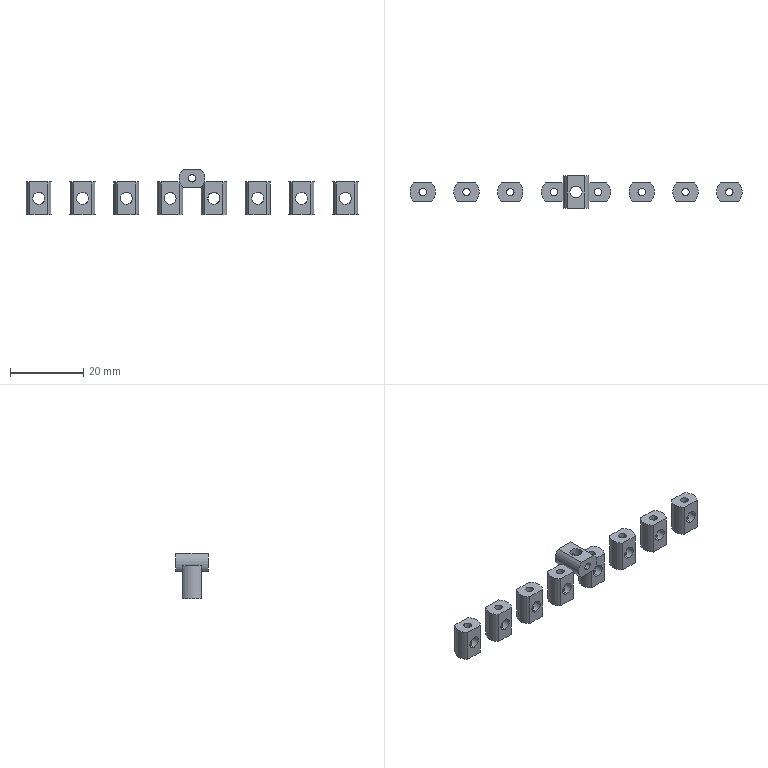CAM job | Mastercam | mm | 15 operations | part box 91 x 9 x 12.5
1. 3D High Speed (Dynamic OptiRough) | 2 - 10C
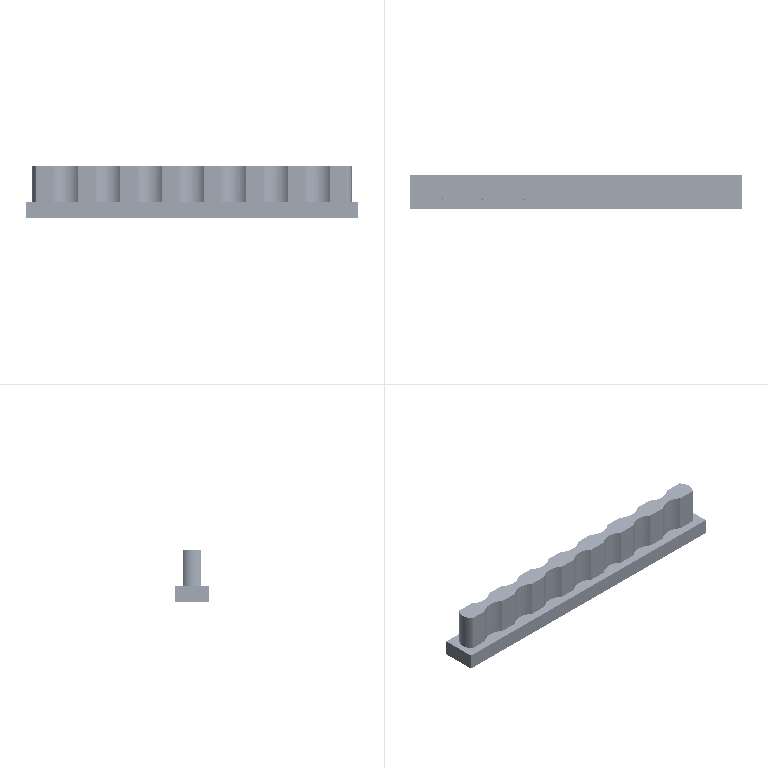2. Facing | 3 - 10J
3. 3D High Speed (Waterline rest passes) | 4 - 4C
4. Contour (2D) | 5 - 4J
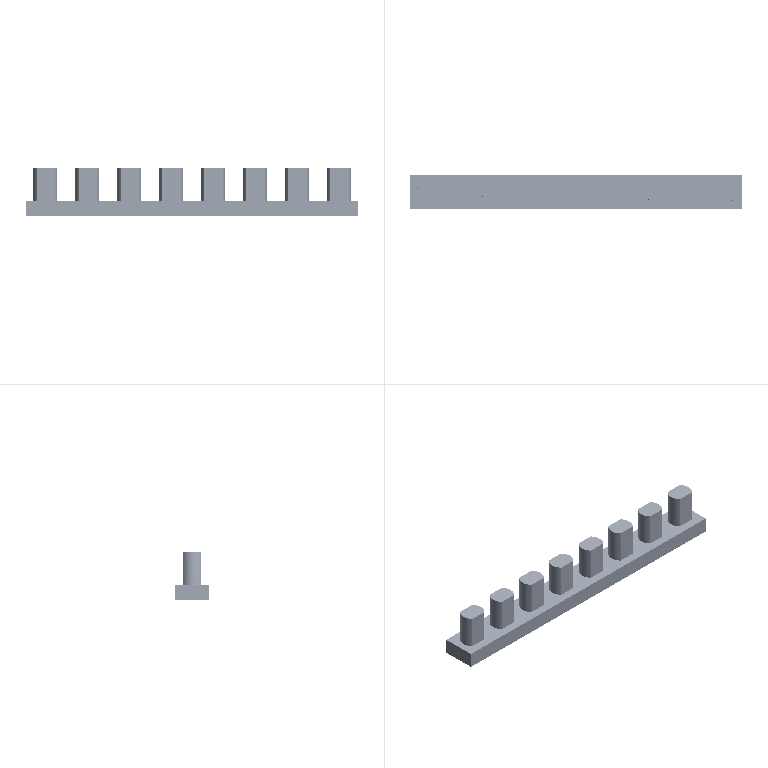5. Drill/Counterbore | 6 - 6 倒角刀
6. Peck Drill | 29 - 2.1 钻头
7. Chamfer Drill | 6 - 6 倒角刀
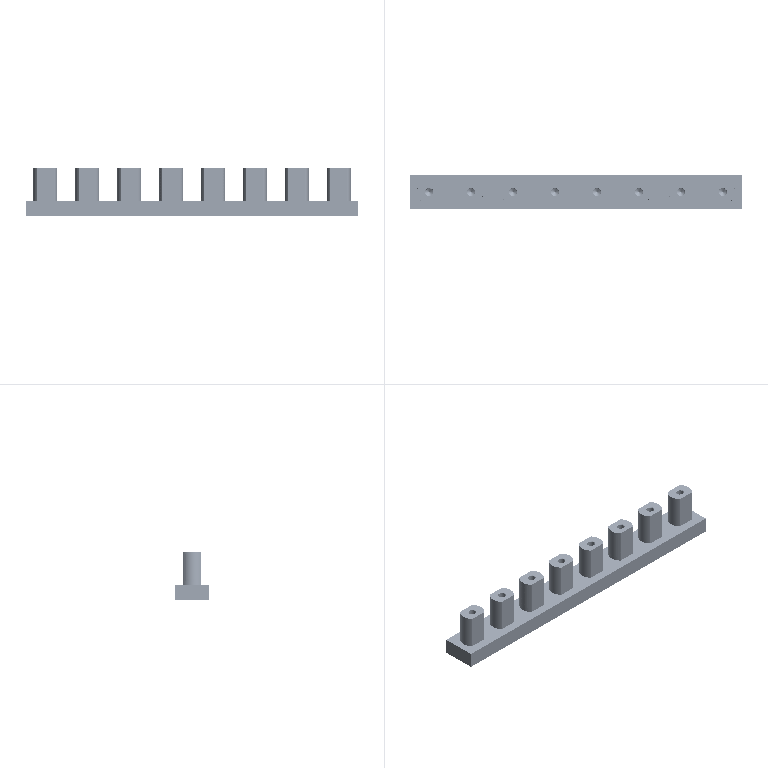8. Contour (2D chamfer) | 6 - 6 倒角刀
9. Drill/Counterbore | 6 - 6 倒角刀
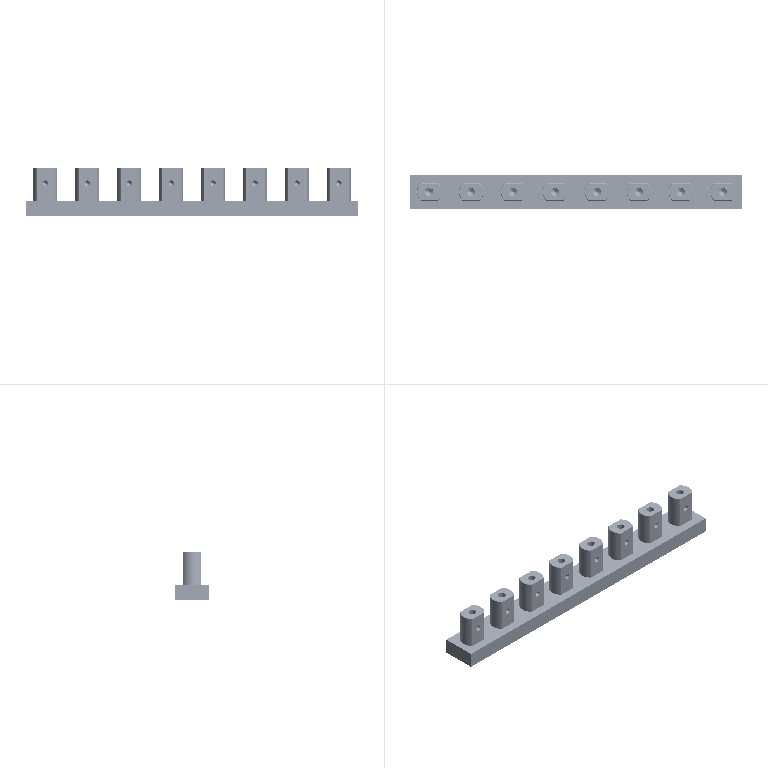10. Peck Drill | 17 - 3.3 钻头
11. Chamfer Drill | 6 - 6 倒角刀
12. Facing | 2 - 10C
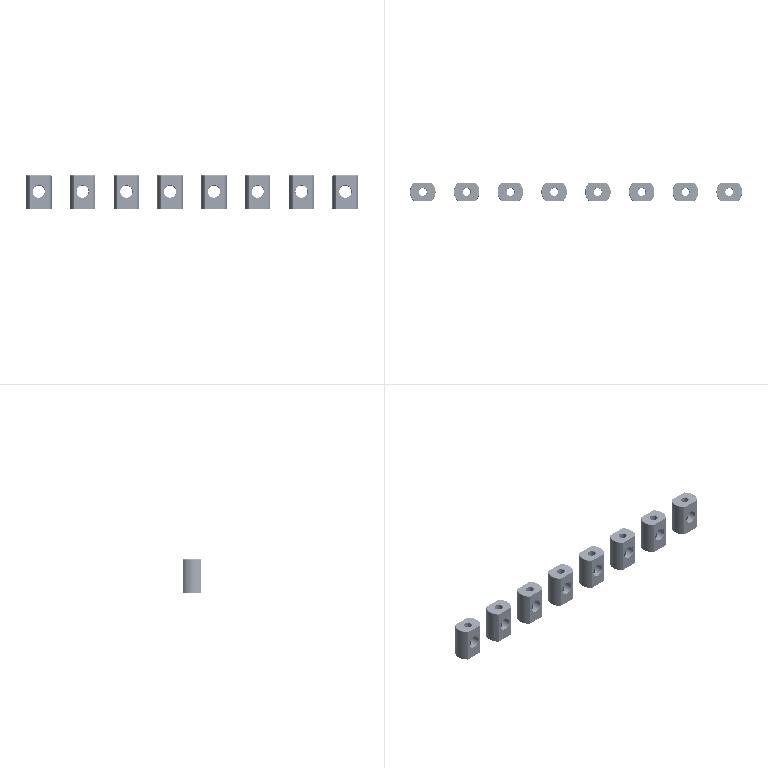13. Facing | 3 - 10J
14. Model Chamfer | 6 - 6 倒角刀
15. Chamfer Drill | 6 - 6 倒角刀